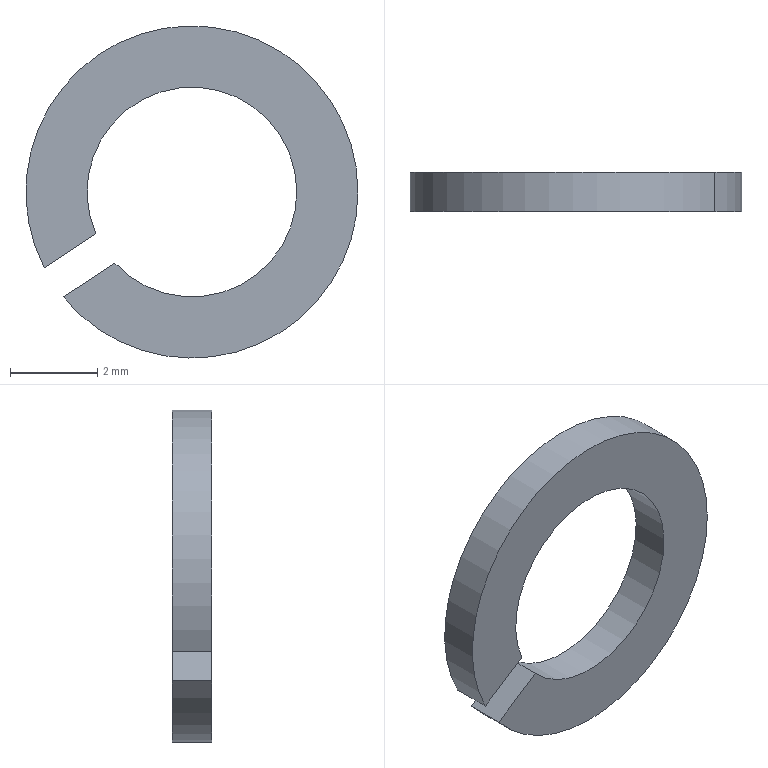Component | SolidWorks | TBN42-4-1 | 1 solid | 7 faces | box 7.6 x 0.9 x 7.6 mm | volume 24 mm3 | plane 4 | cylinder 3 | commonest cylinder face diameters 7.6 x2 4.8 x1
build123d program:
from build123d import *
from build123d.topology import SkipClean

# Parameters (mm, degrees)
SKETCH1_W               = 1.75
SKETCH1_H               = 0.9
REVOLVE1_ANGLE          = 180
SKETCH2_W               = 1.75
SKETCH2_H               = 0.9
REVOLVE2_ANGLE          = 180
CUT_EXTRUDE1_DEPTH      = 7.6
CUT_EXTRUDE1_DEPTH_BACK = 7.6
SKETCH3_W               = 7.6
SKETCH3_H               = 0.8
SKETCH4_R               = 2.4
CUT_EXTRUDE2_DEPTH      = 6.449


with BuildPart() as part:
    # Sketch1 → Revolve1 (revolve)
    with BuildSketch(Plane(origin=(0, 0, 0), x_dir=(1, 0, 0), z_dir=(0, 1, 0))):
        with Locations((2.925, -0.45)):
            Rectangle(SKETCH1_W, SKETCH1_H)
    revolve(axis=Axis((0, 0, 0.9), (0, 0, -1)), revolution_arc=REVOLVE1_ANGLE)

    # Sketch2 → Revolve2 (revolve)
    with SkipClean():  # the faces are left unmerged after this step: merging them gives an invalid solid
        with BuildSketch(Plane(origin=(0, 0, 0), x_dir=(1, 0, 0), z_dir=(0, 1, 0))):
            with Locations((2.925, -0.45)):
                Rectangle(SKETCH2_W, SKETCH2_H)
        revolve(axis=Axis((0, 0, 0.9), (0, 0, 1)), revolution_arc=REVOLVE2_ANGLE)

    # Sketch3 → Cut-Extrude1 (cut, two sides: drawn at the far end of the back side and taken through both)
    with BuildSketch(Plane.XY.offset(-CUT_EXTRUDE1_DEPTH_BACK)):
        with Locations((-3.8, 0)):
            Rectangle(SKETCH3_W, SKETCH3_H)
    extrude(amount=CUT_EXTRUDE1_DEPTH + CUT_EXTRUDE1_DEPTH_BACK, mode=Mode.SUBTRACT)

    # Sketch4 → Cut-Extrude2 (cut, through all)
    with BuildSketch(Plane.XY):
        Circle(SKETCH4_R)
    extrude(amount=CUT_EXTRUDE2_DEPTH, mode=Mode.SUBTRACT)


solid = part.part

# Placed as in the assembly
solid = solid.moved(Location((-187.536, 78.75, 217.788), (90, 0, 33.158)))